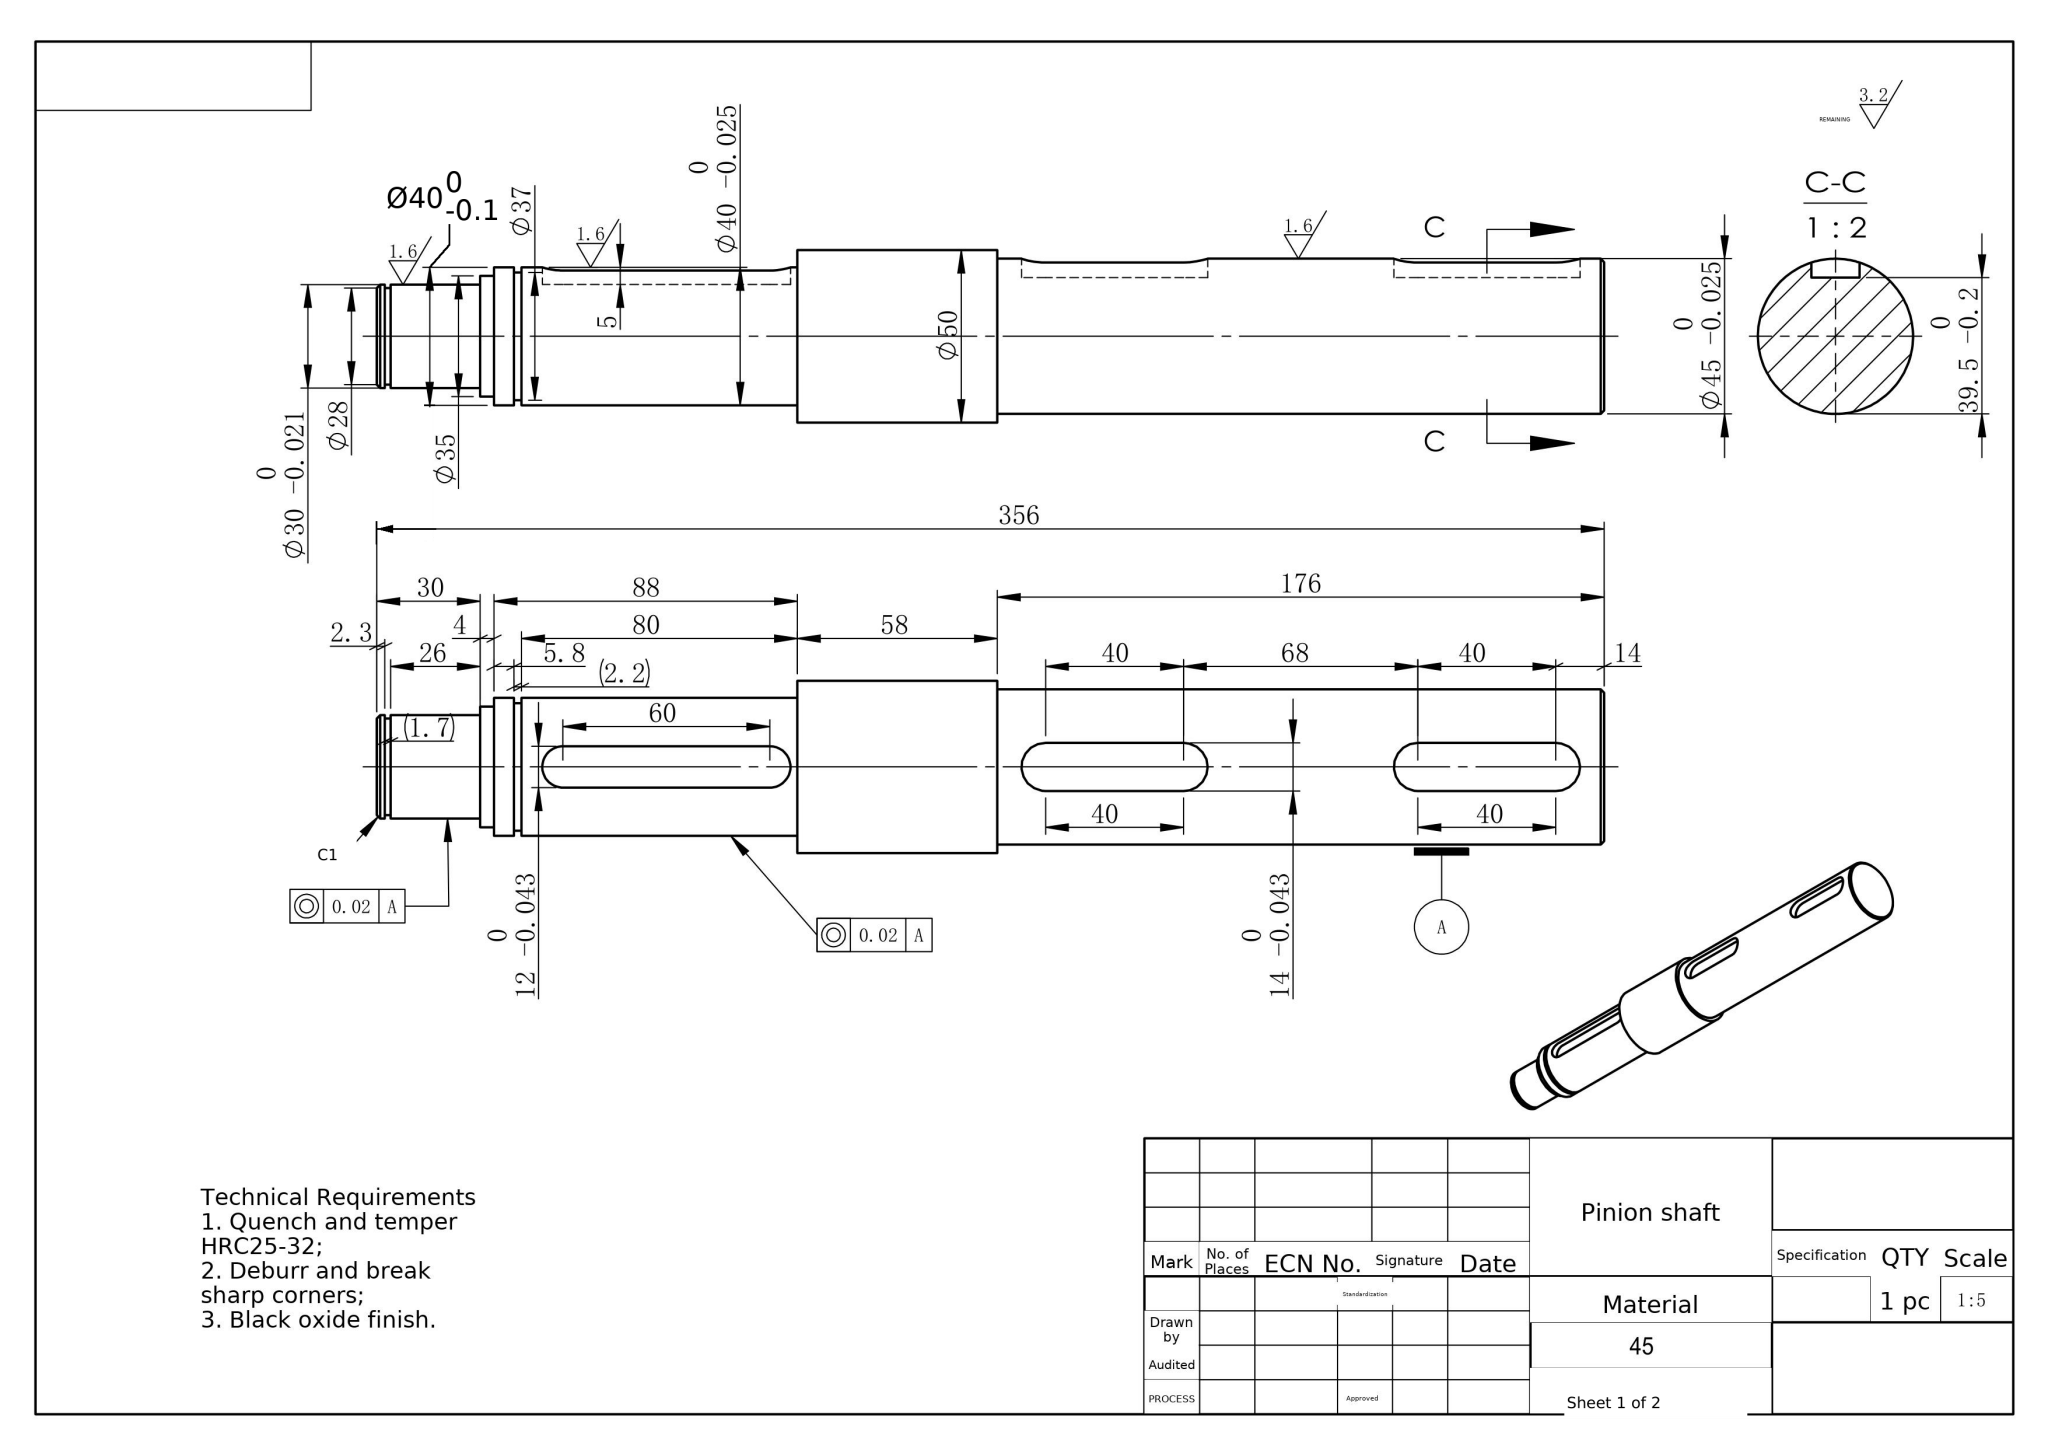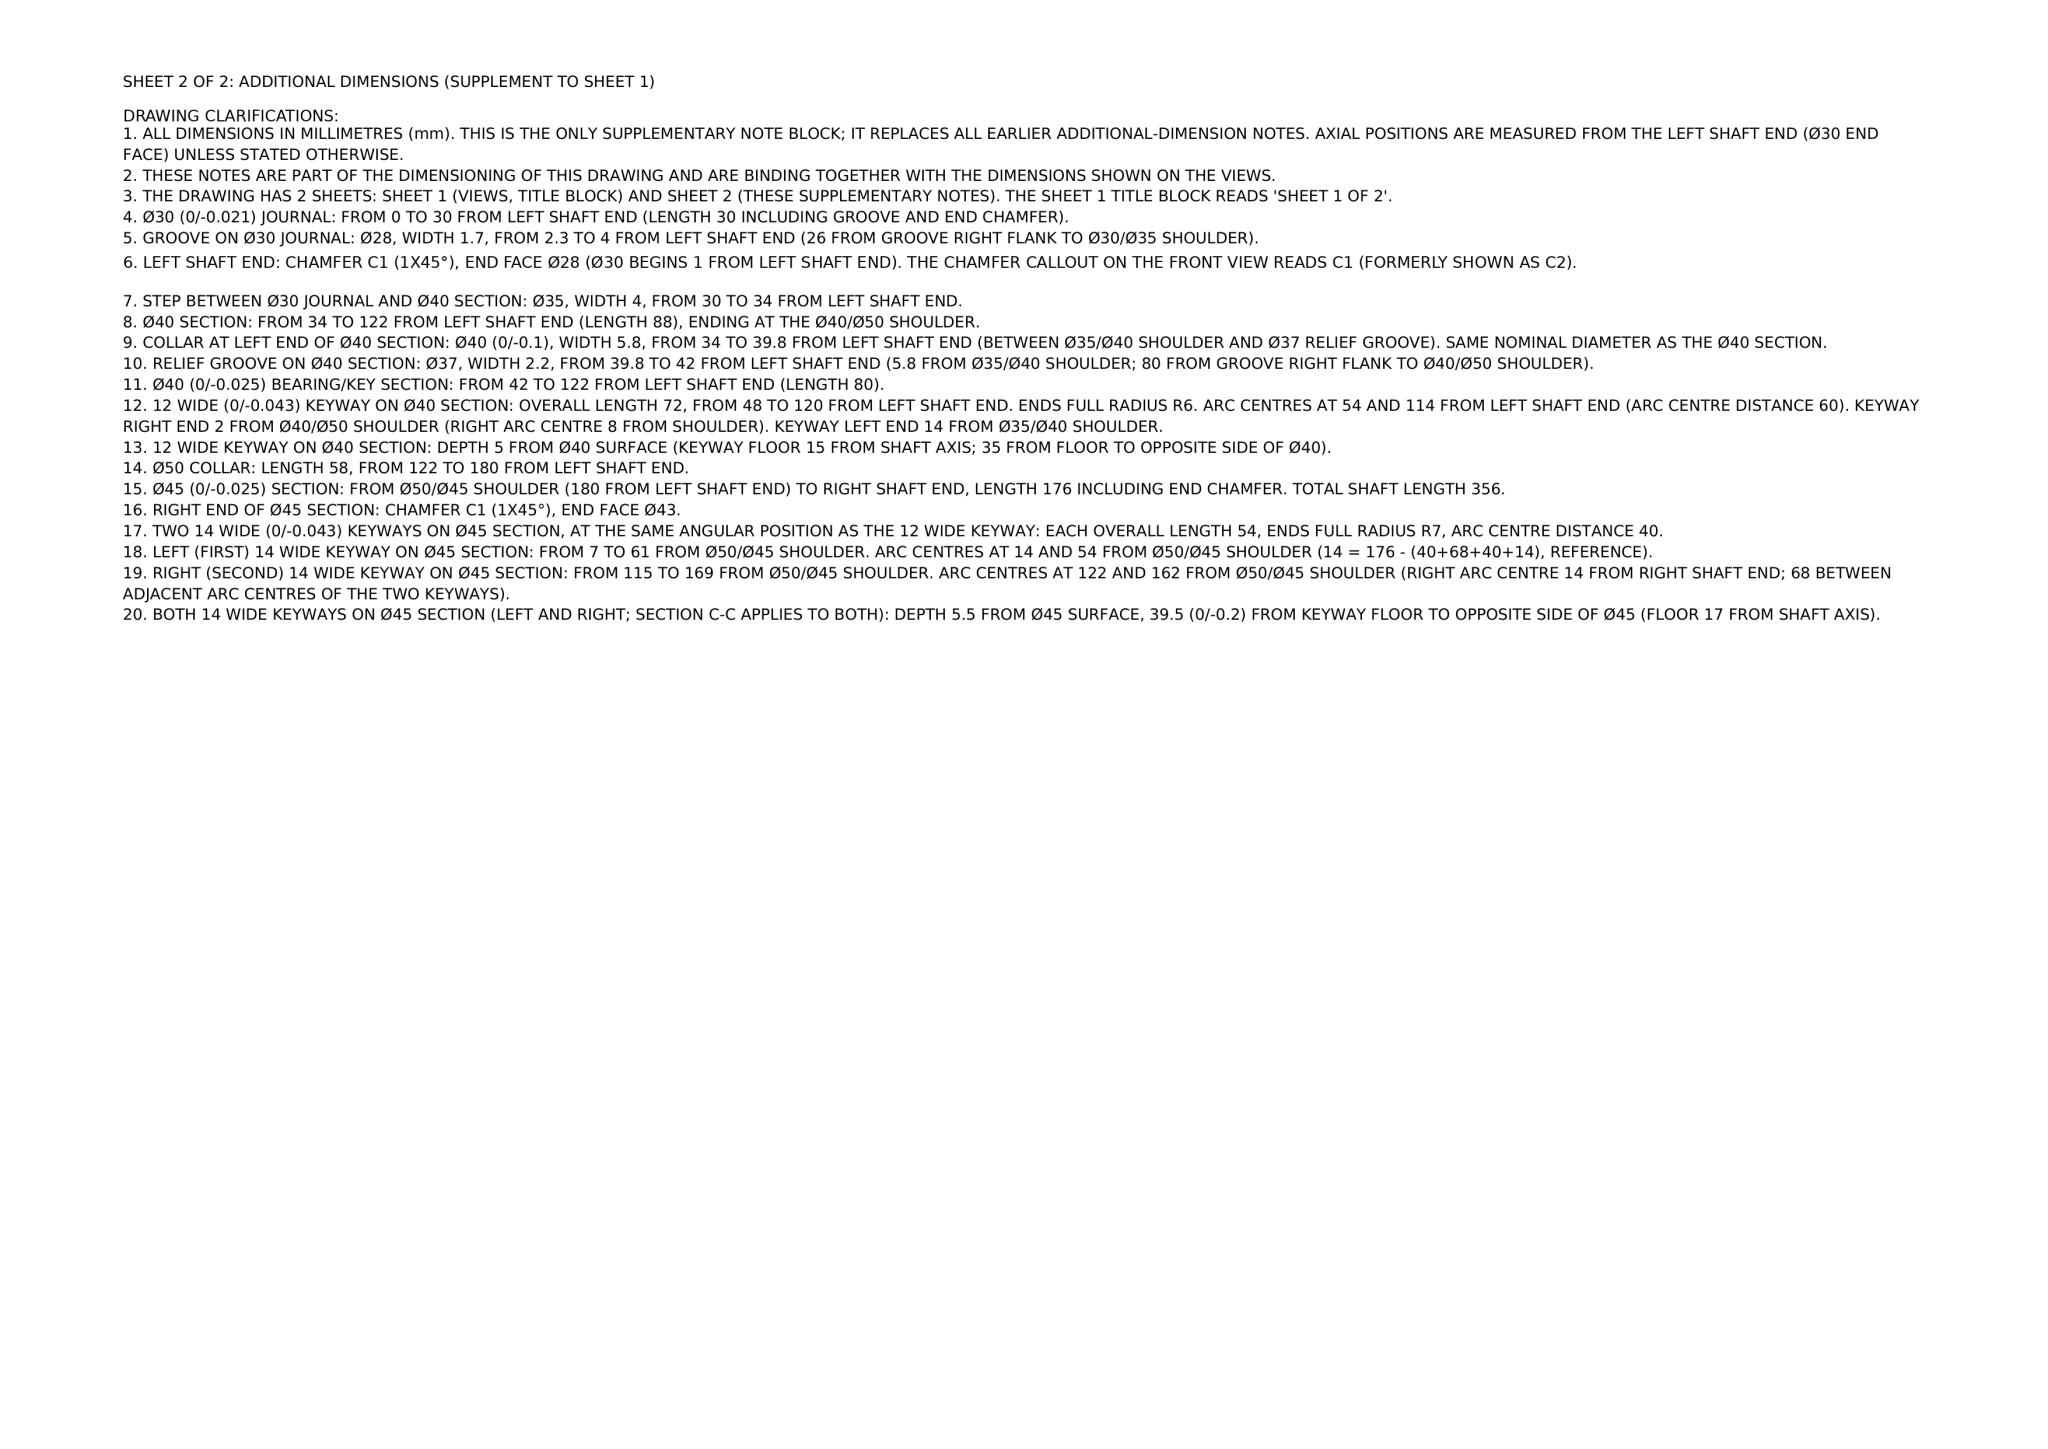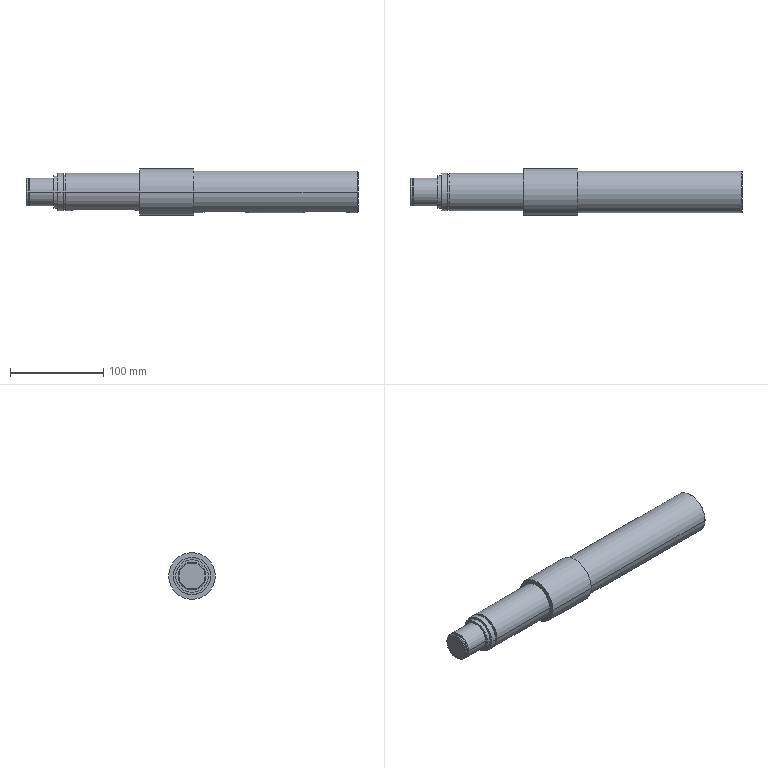Part | NX | mm | 1 solid | 50 faces | box 356 x 50 x 50 mm | volume 517491 mm3 | cylinder 27 | plane 19 | cone 4 | commonest cylinder face diameters 14 x6 40 x4 30 x4 12 x3 35 x2 37 x2 50 x2 45 x2